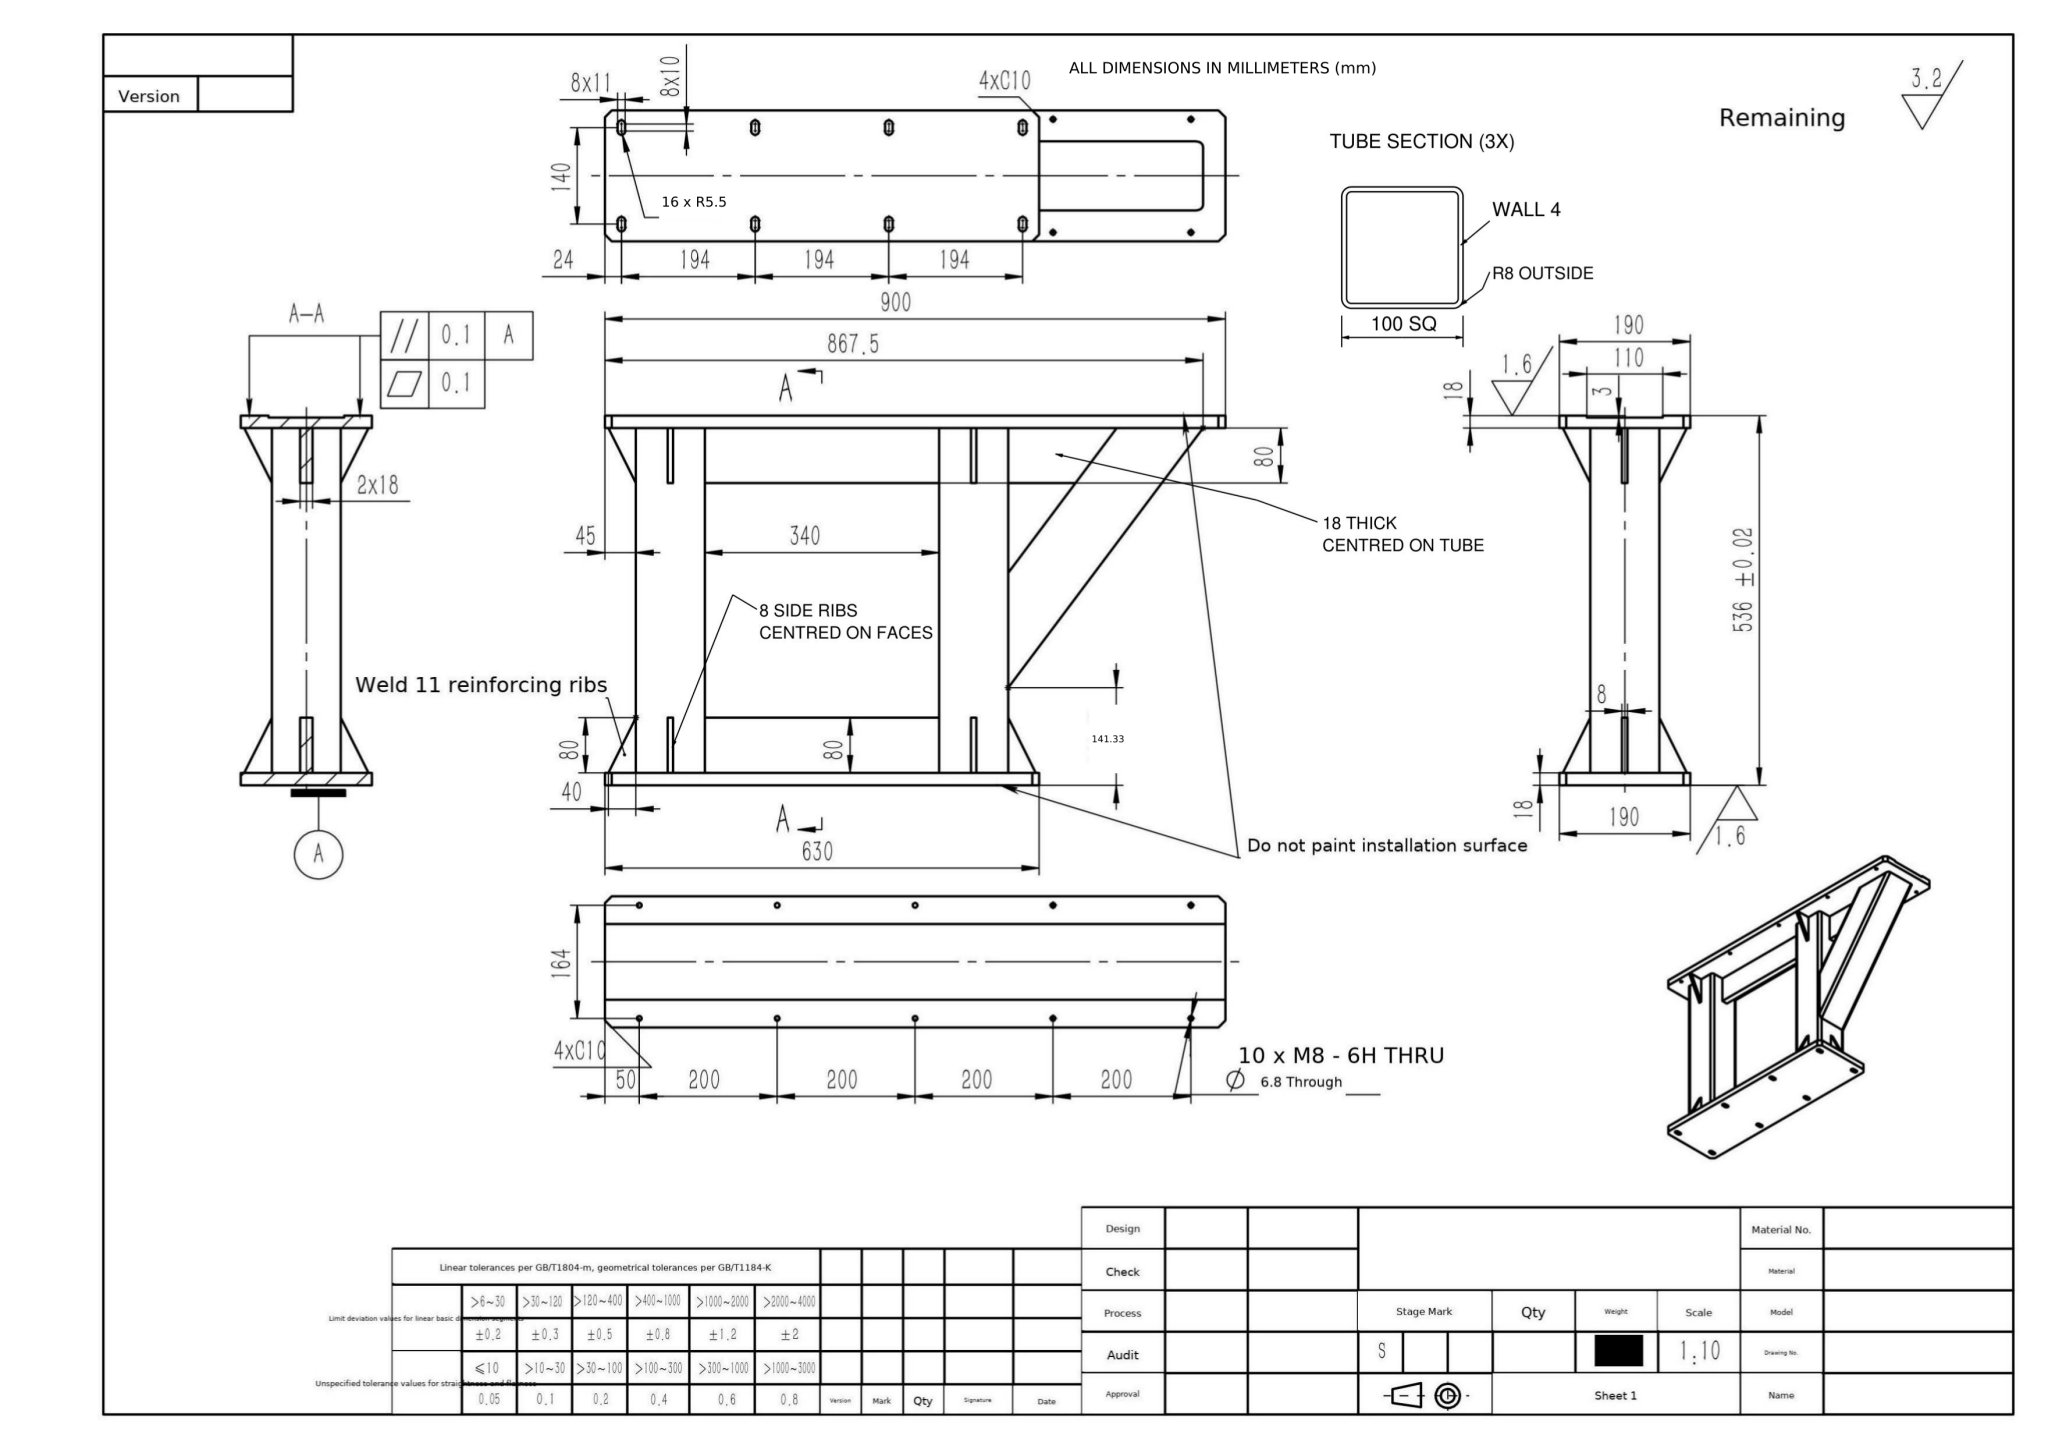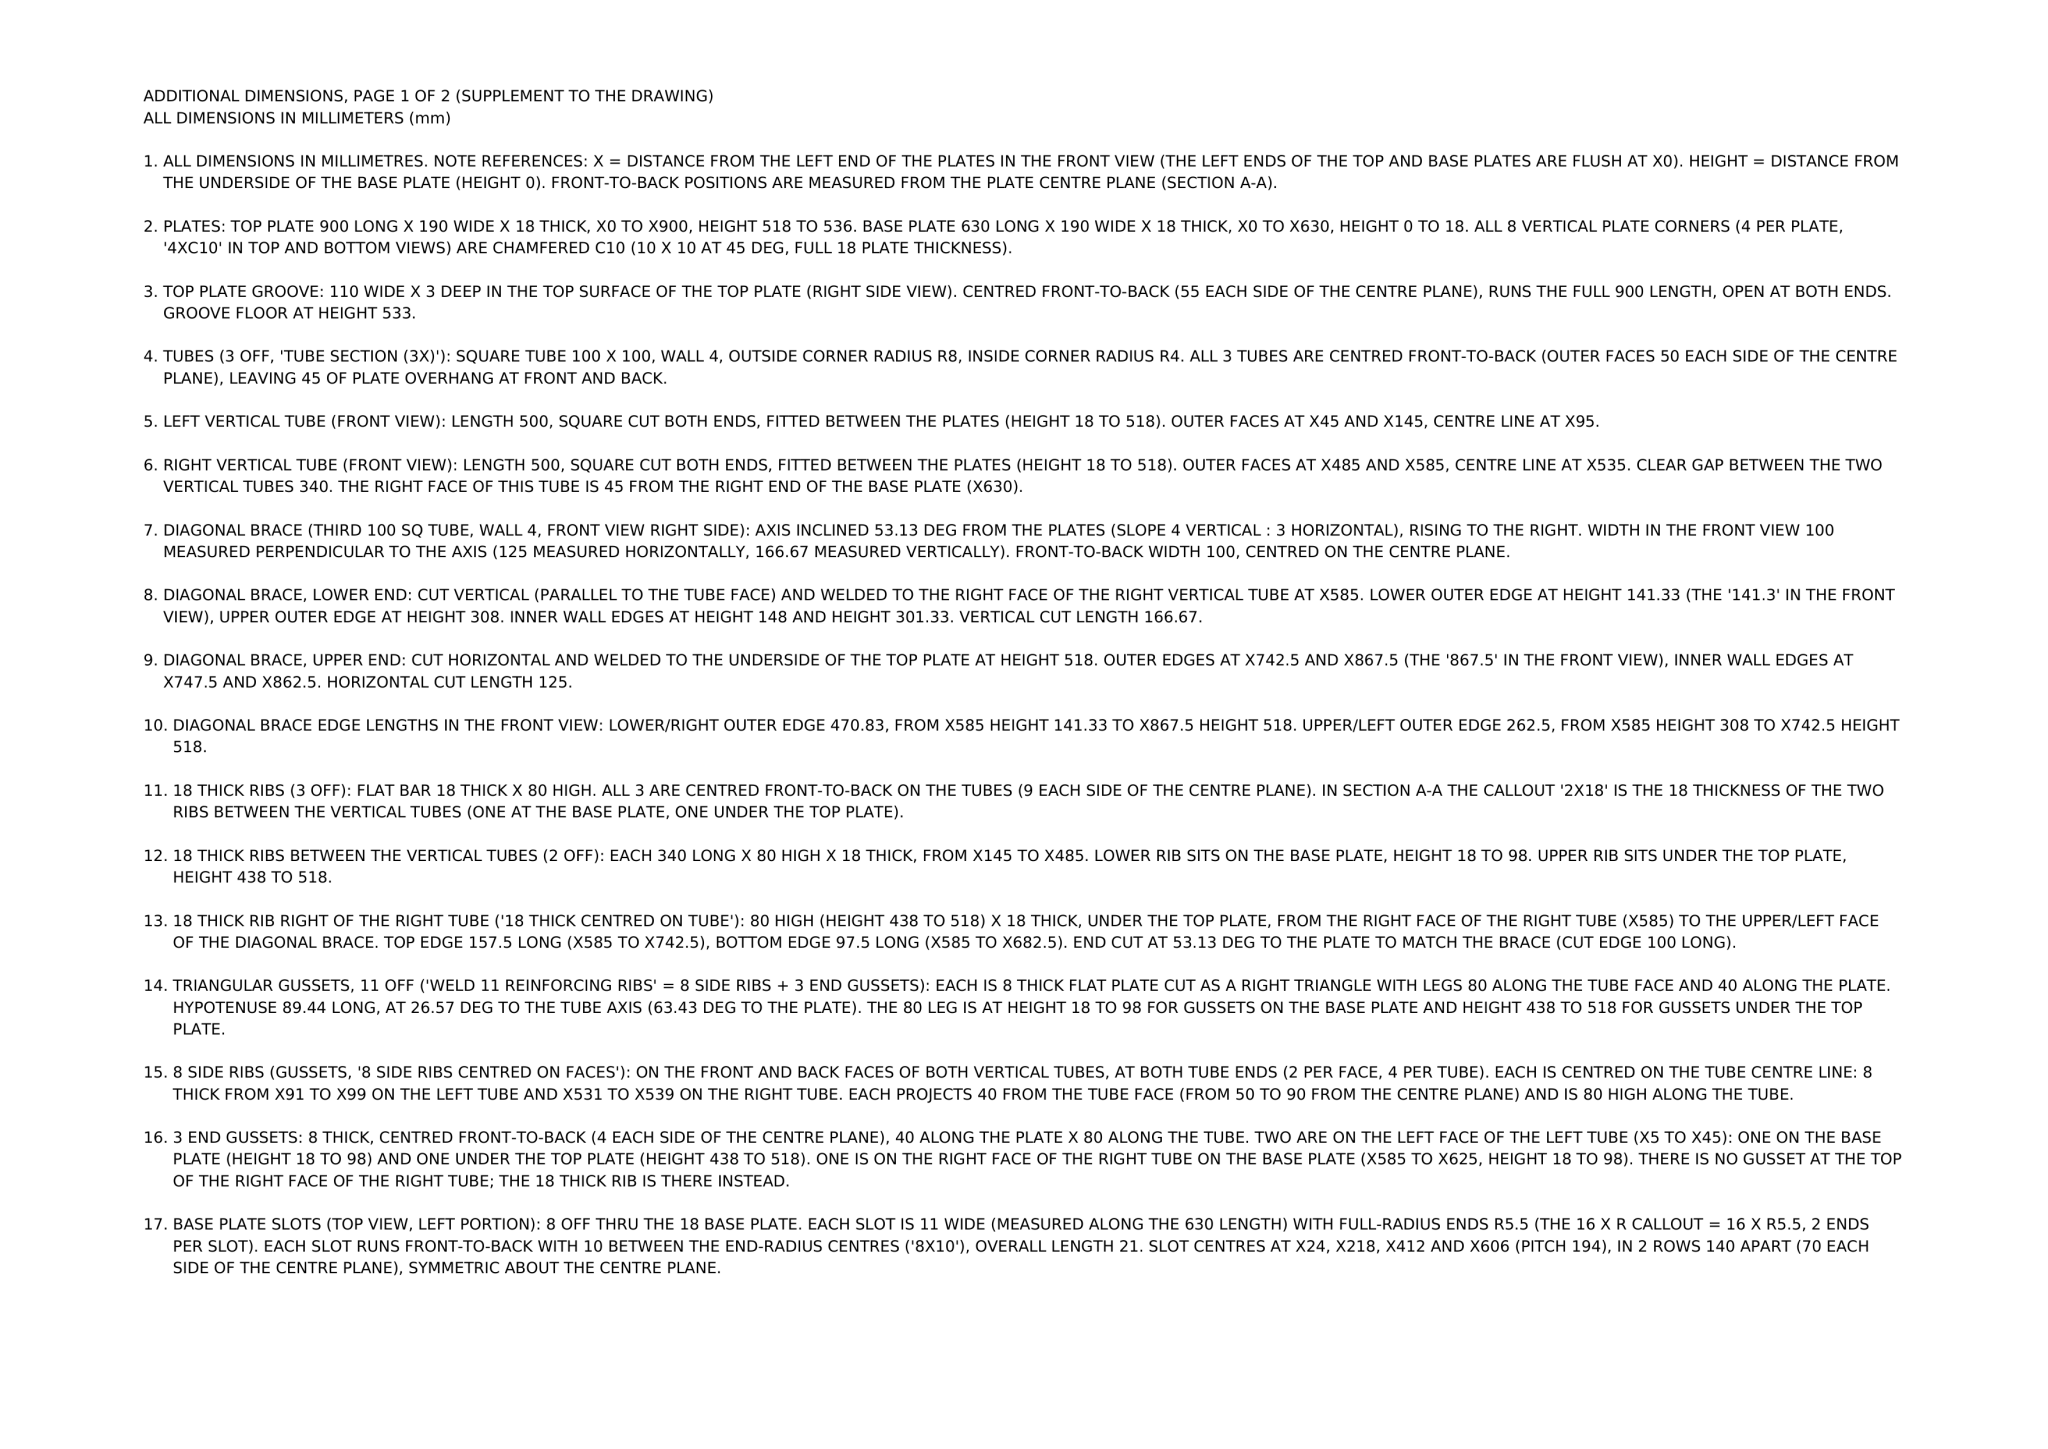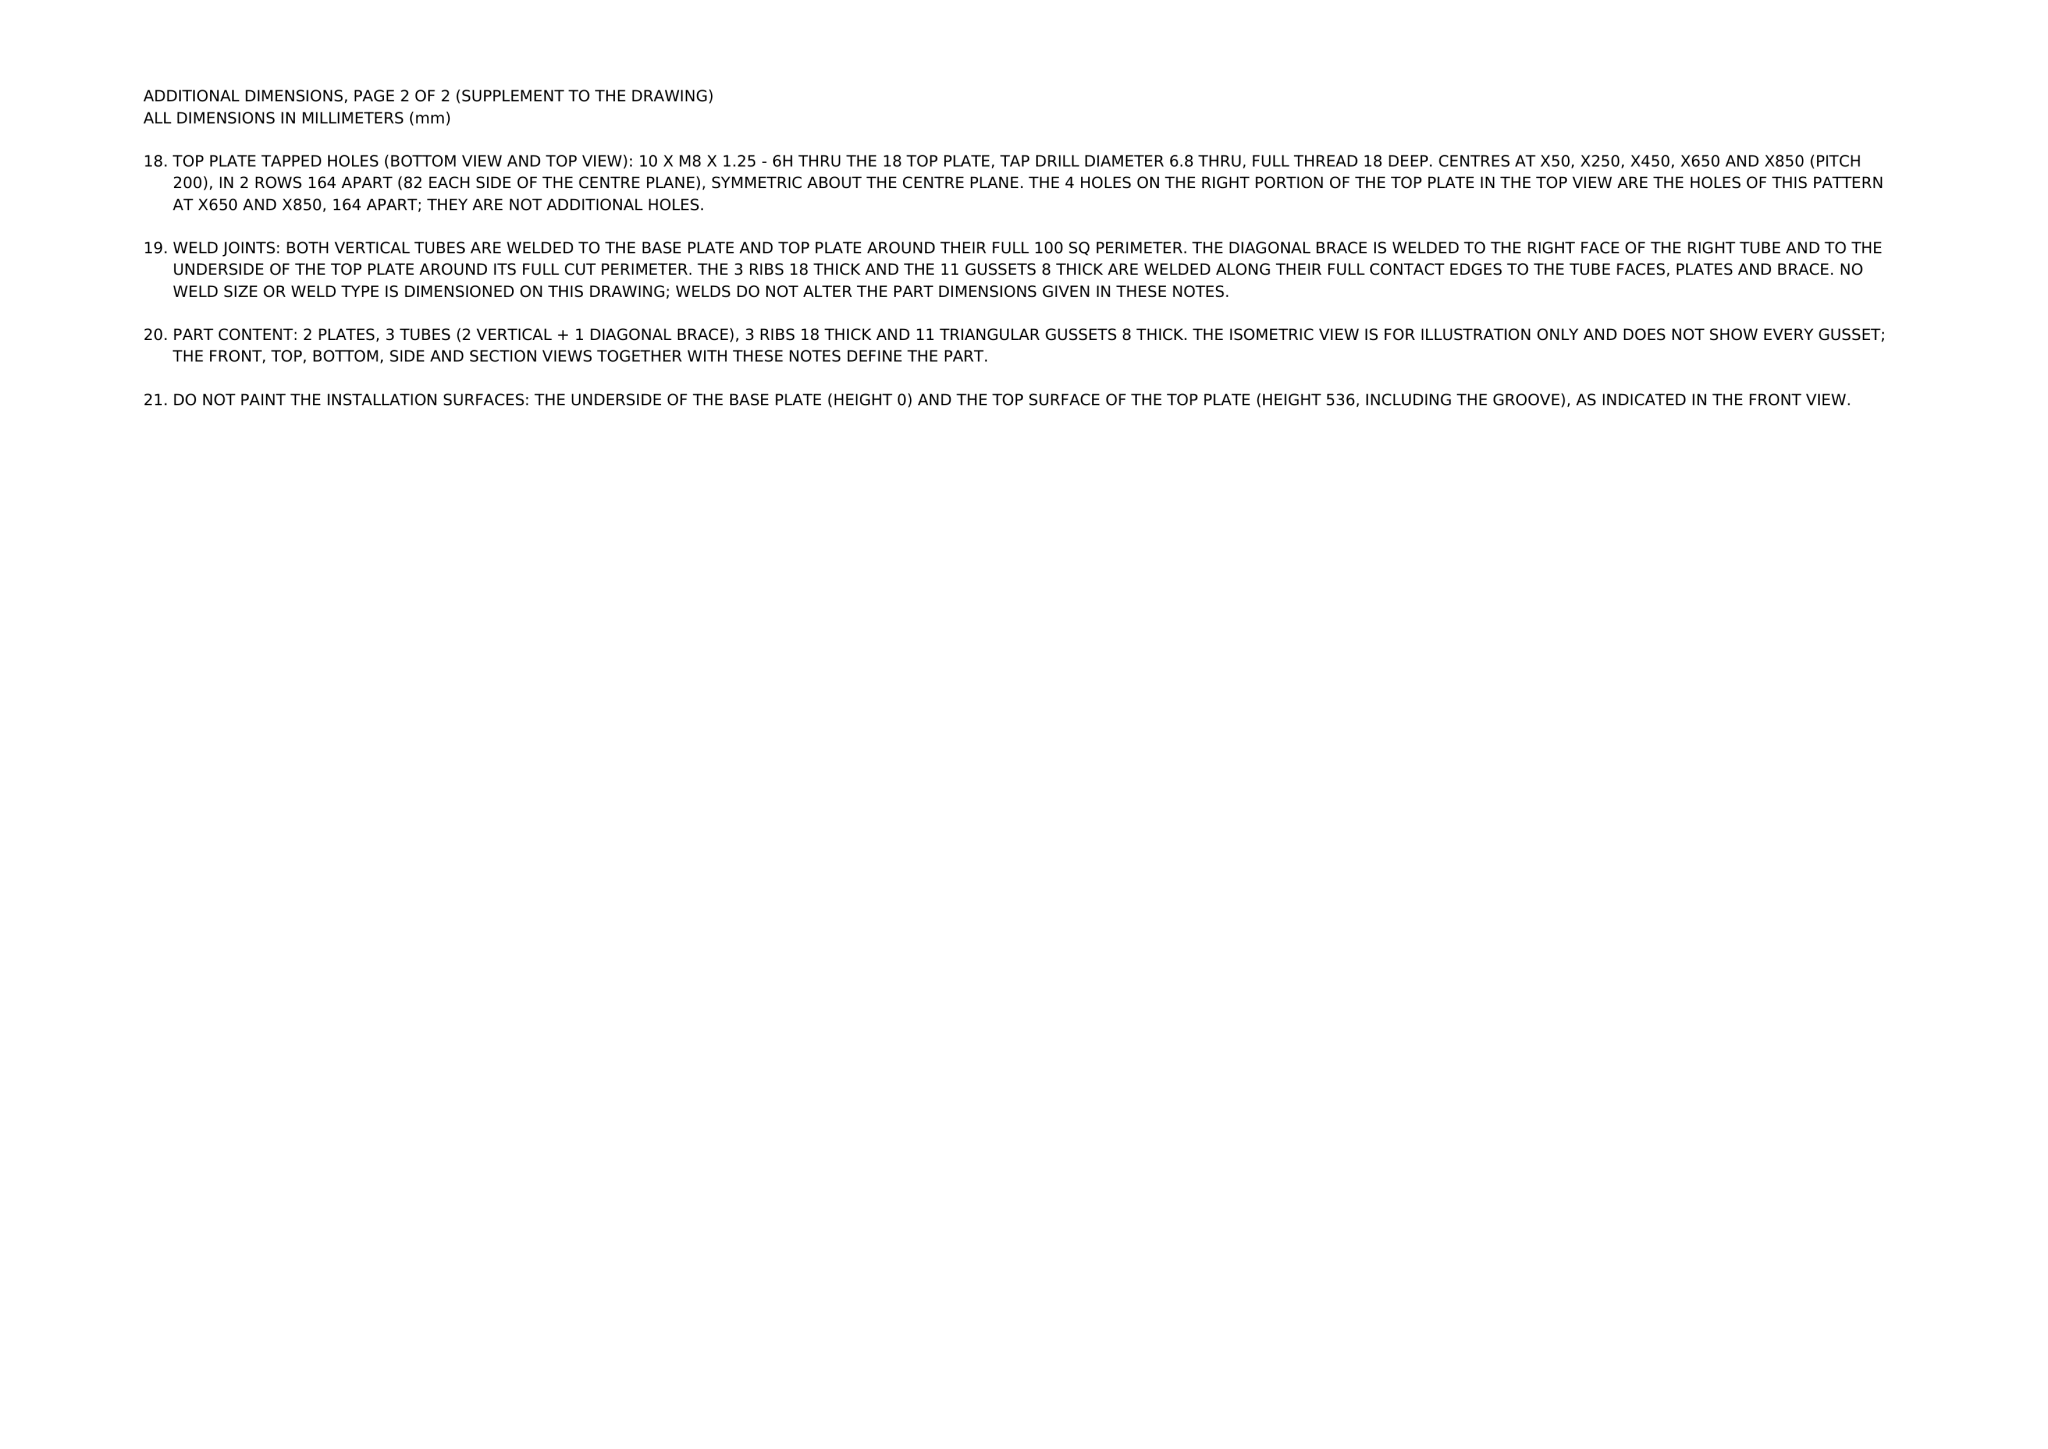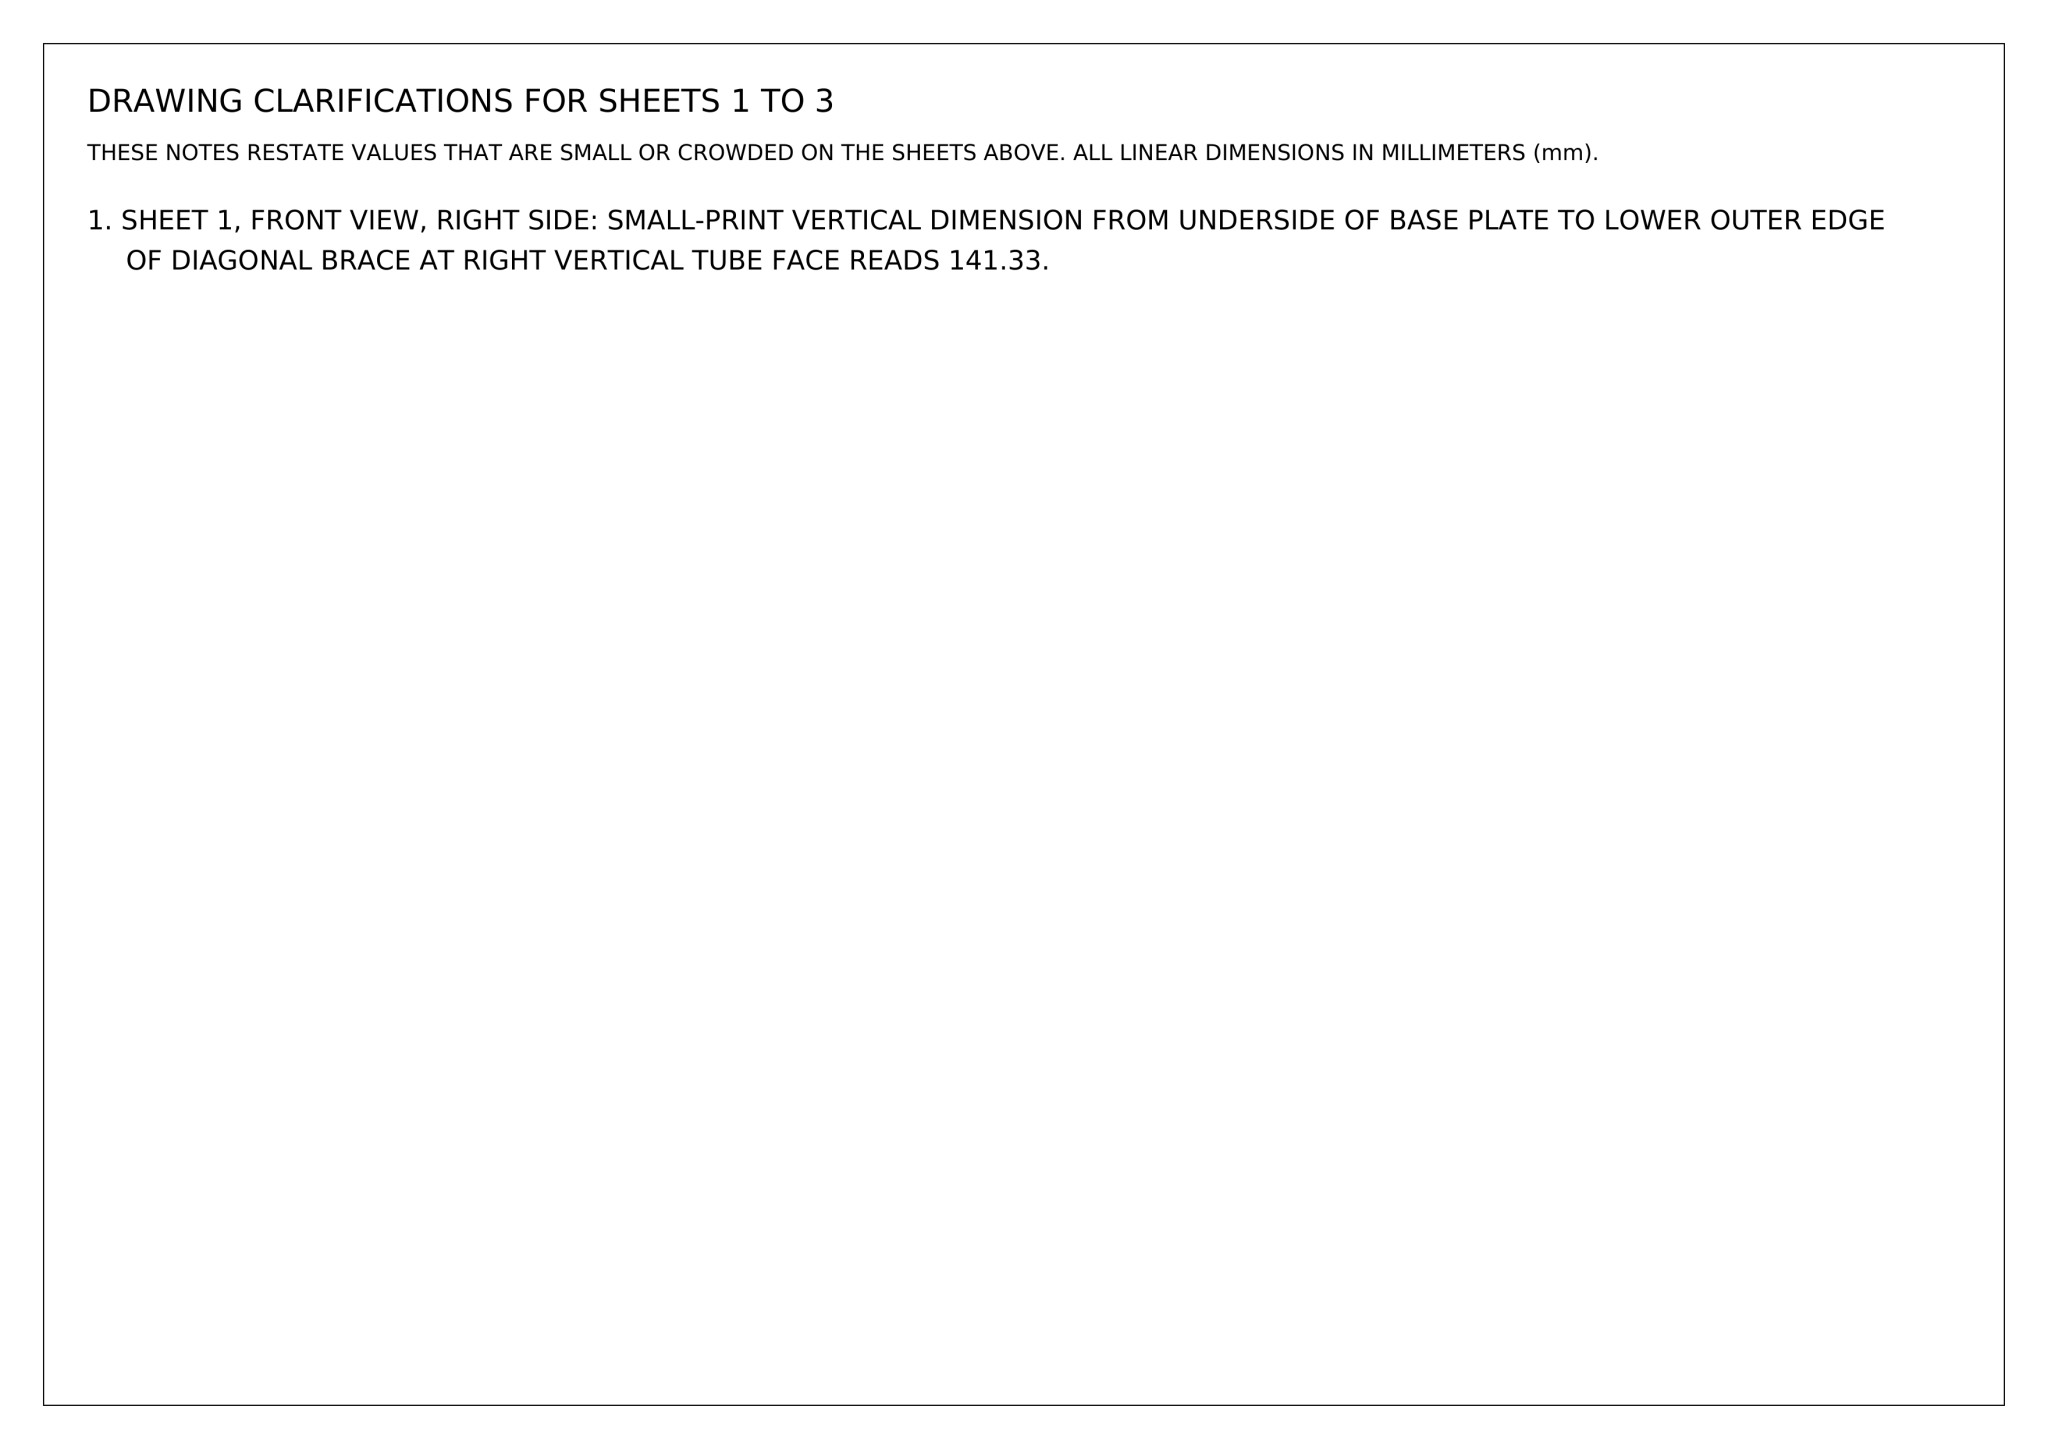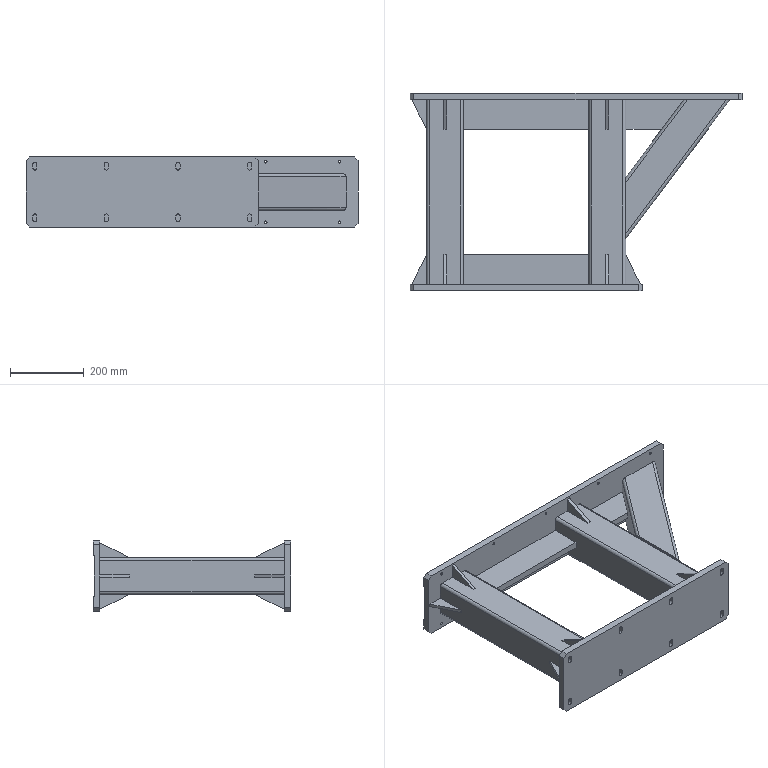Part | NX | mm | 1 solid | 175 faces | box 900 x 536 x 190 mm | volume 8238827 mm3 | plane 115 | cylinder 60 | commonest cylinder face diameters 6.8 x20 11 x16 16 x12 8 x12